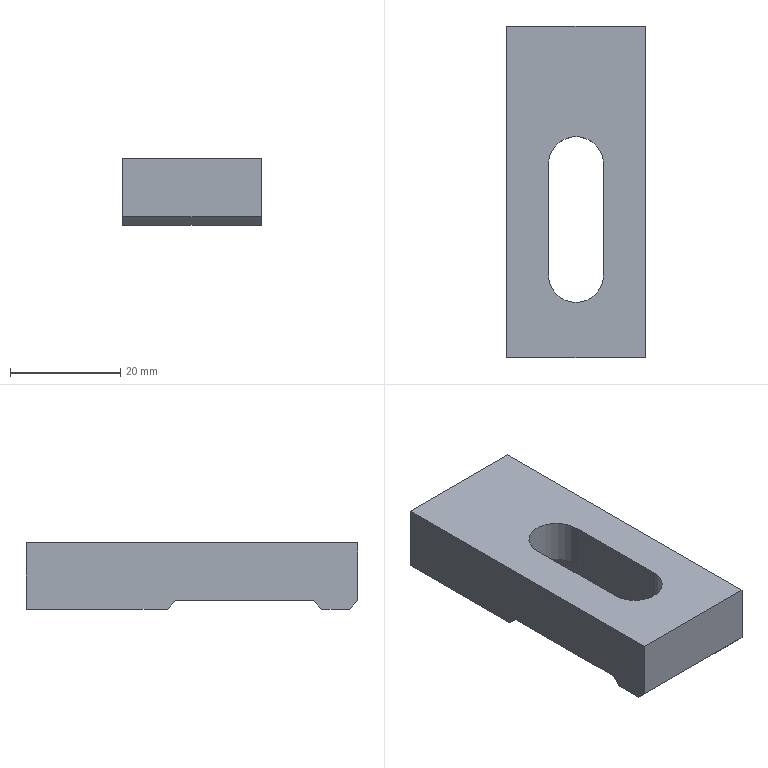Component | NX | MOV_CLAMP_PLATE | 1 solid | 18 faces | volume 13133 mm3 | plane 16 | cylinder 2 | commonest cylinder face diameters 10 x2